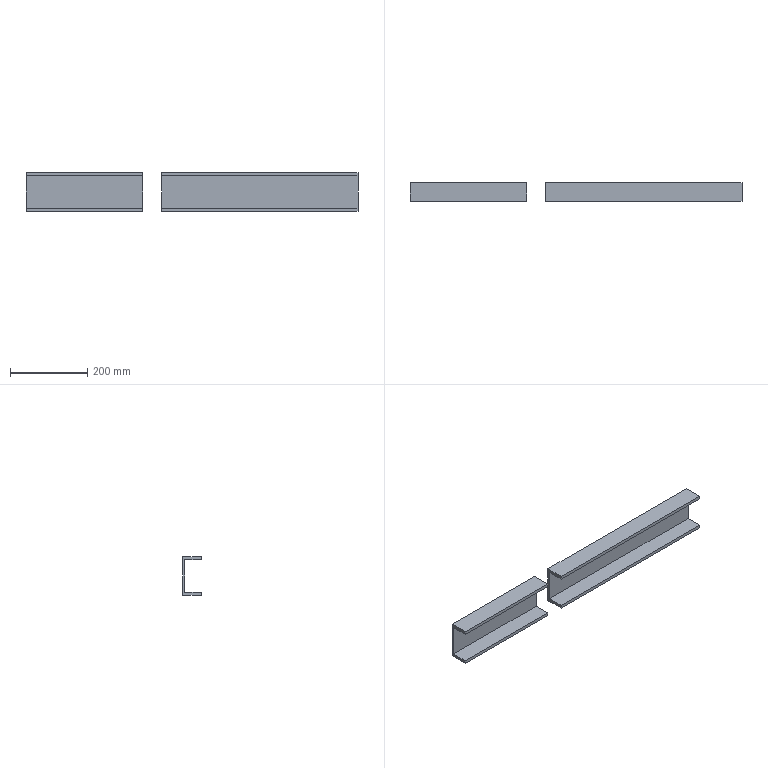Component | NX | CHUNSHUIJINCAO_CAOGANG3 | 2 solids | 20 faces | volume 1016023 mm3 | plane 20